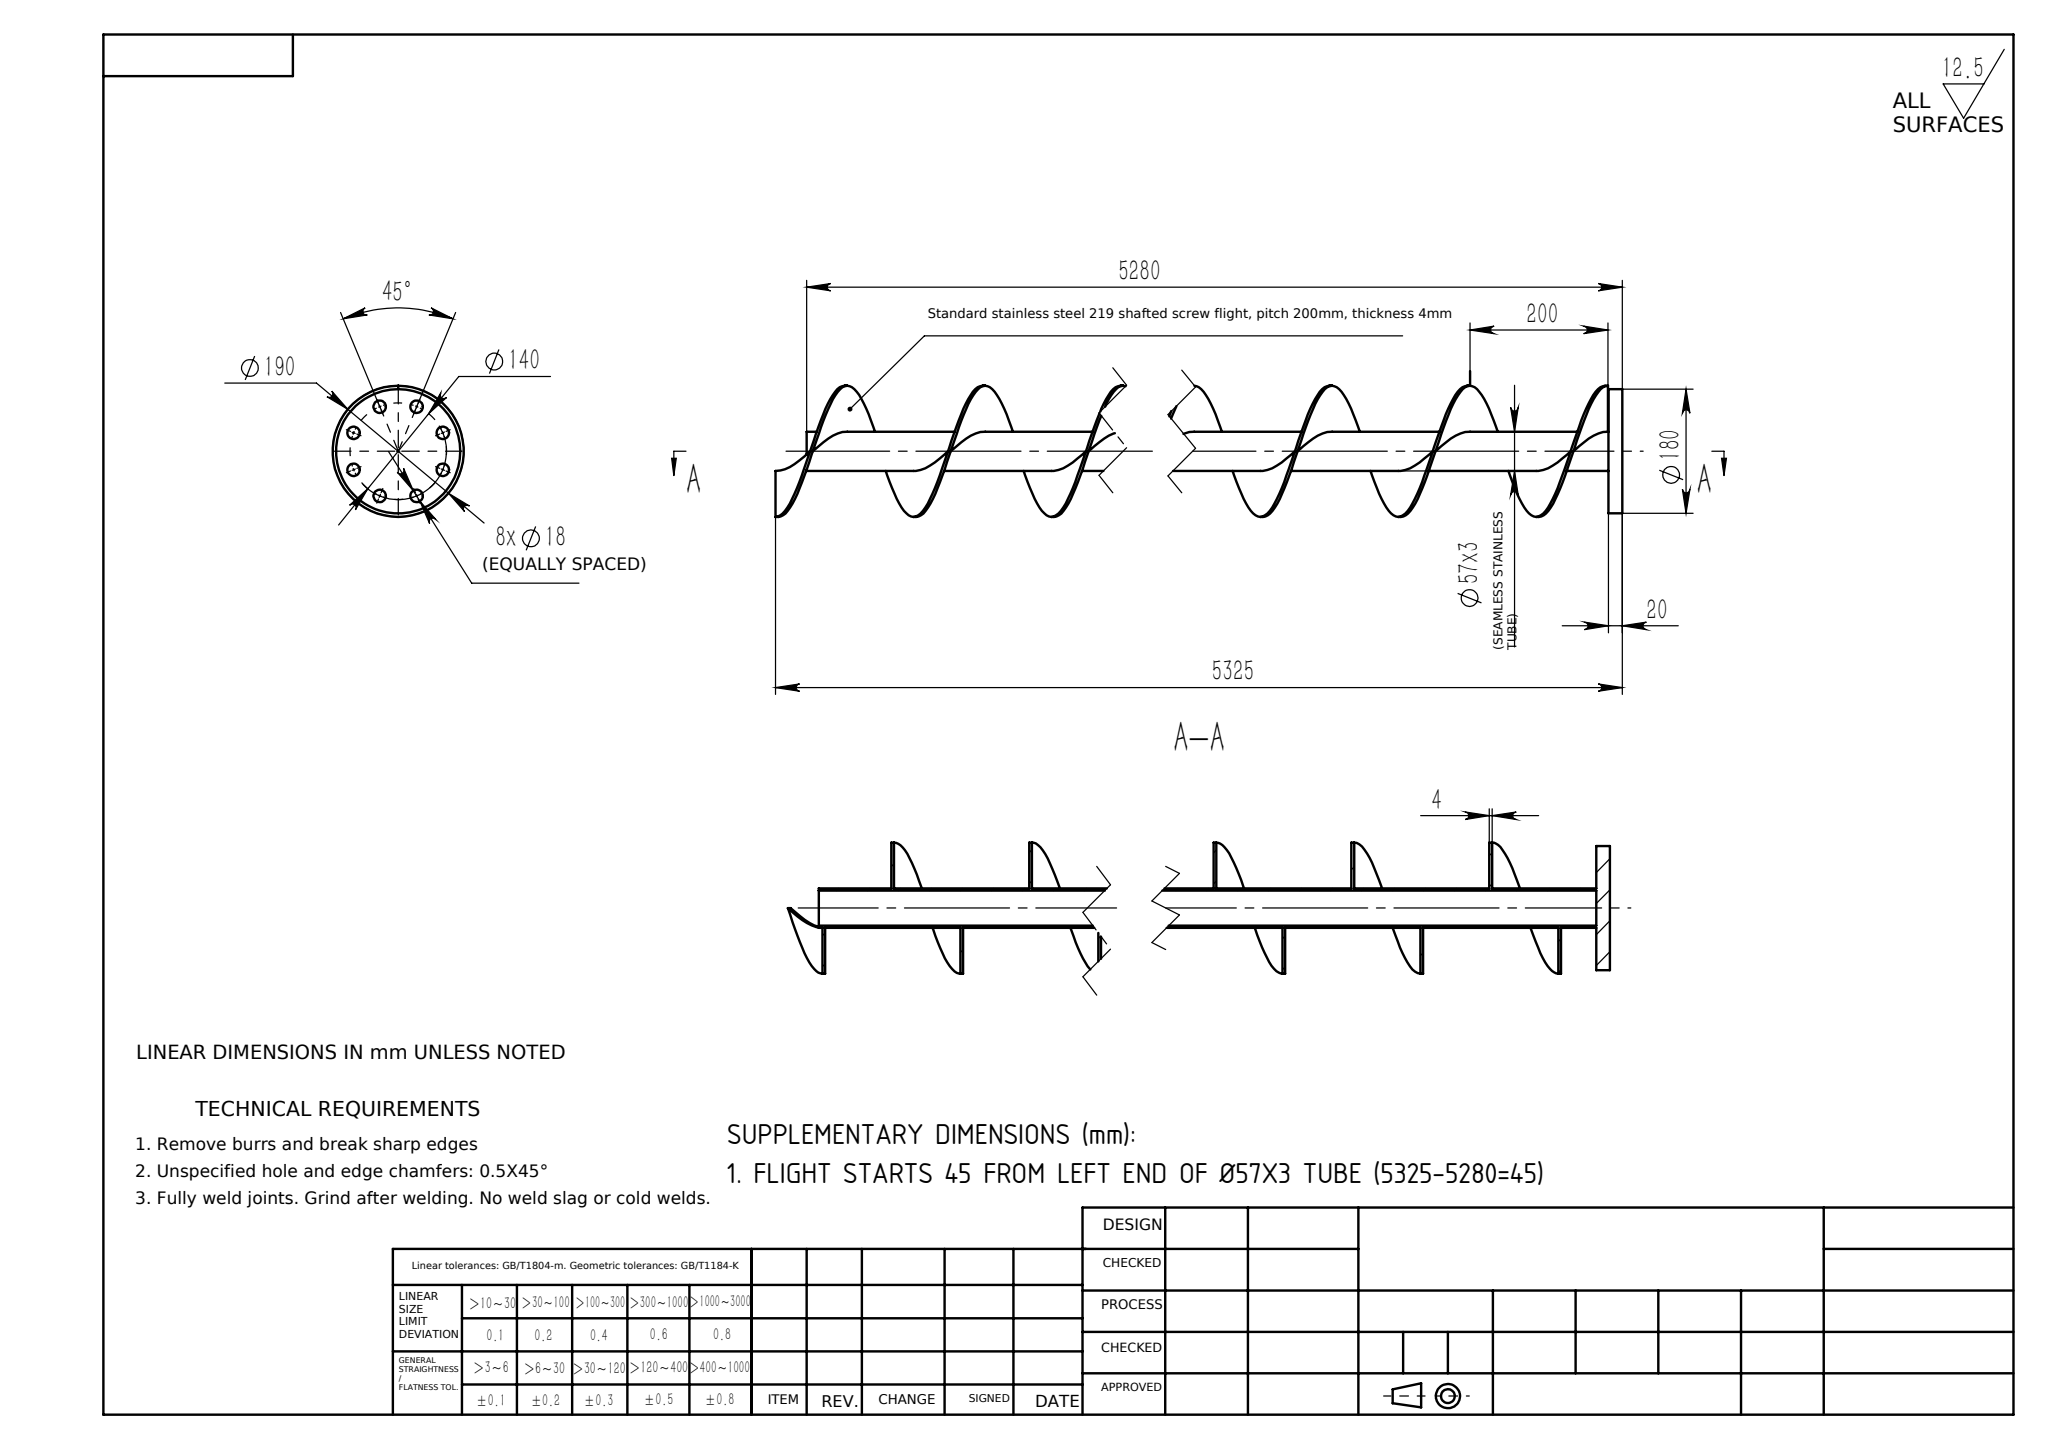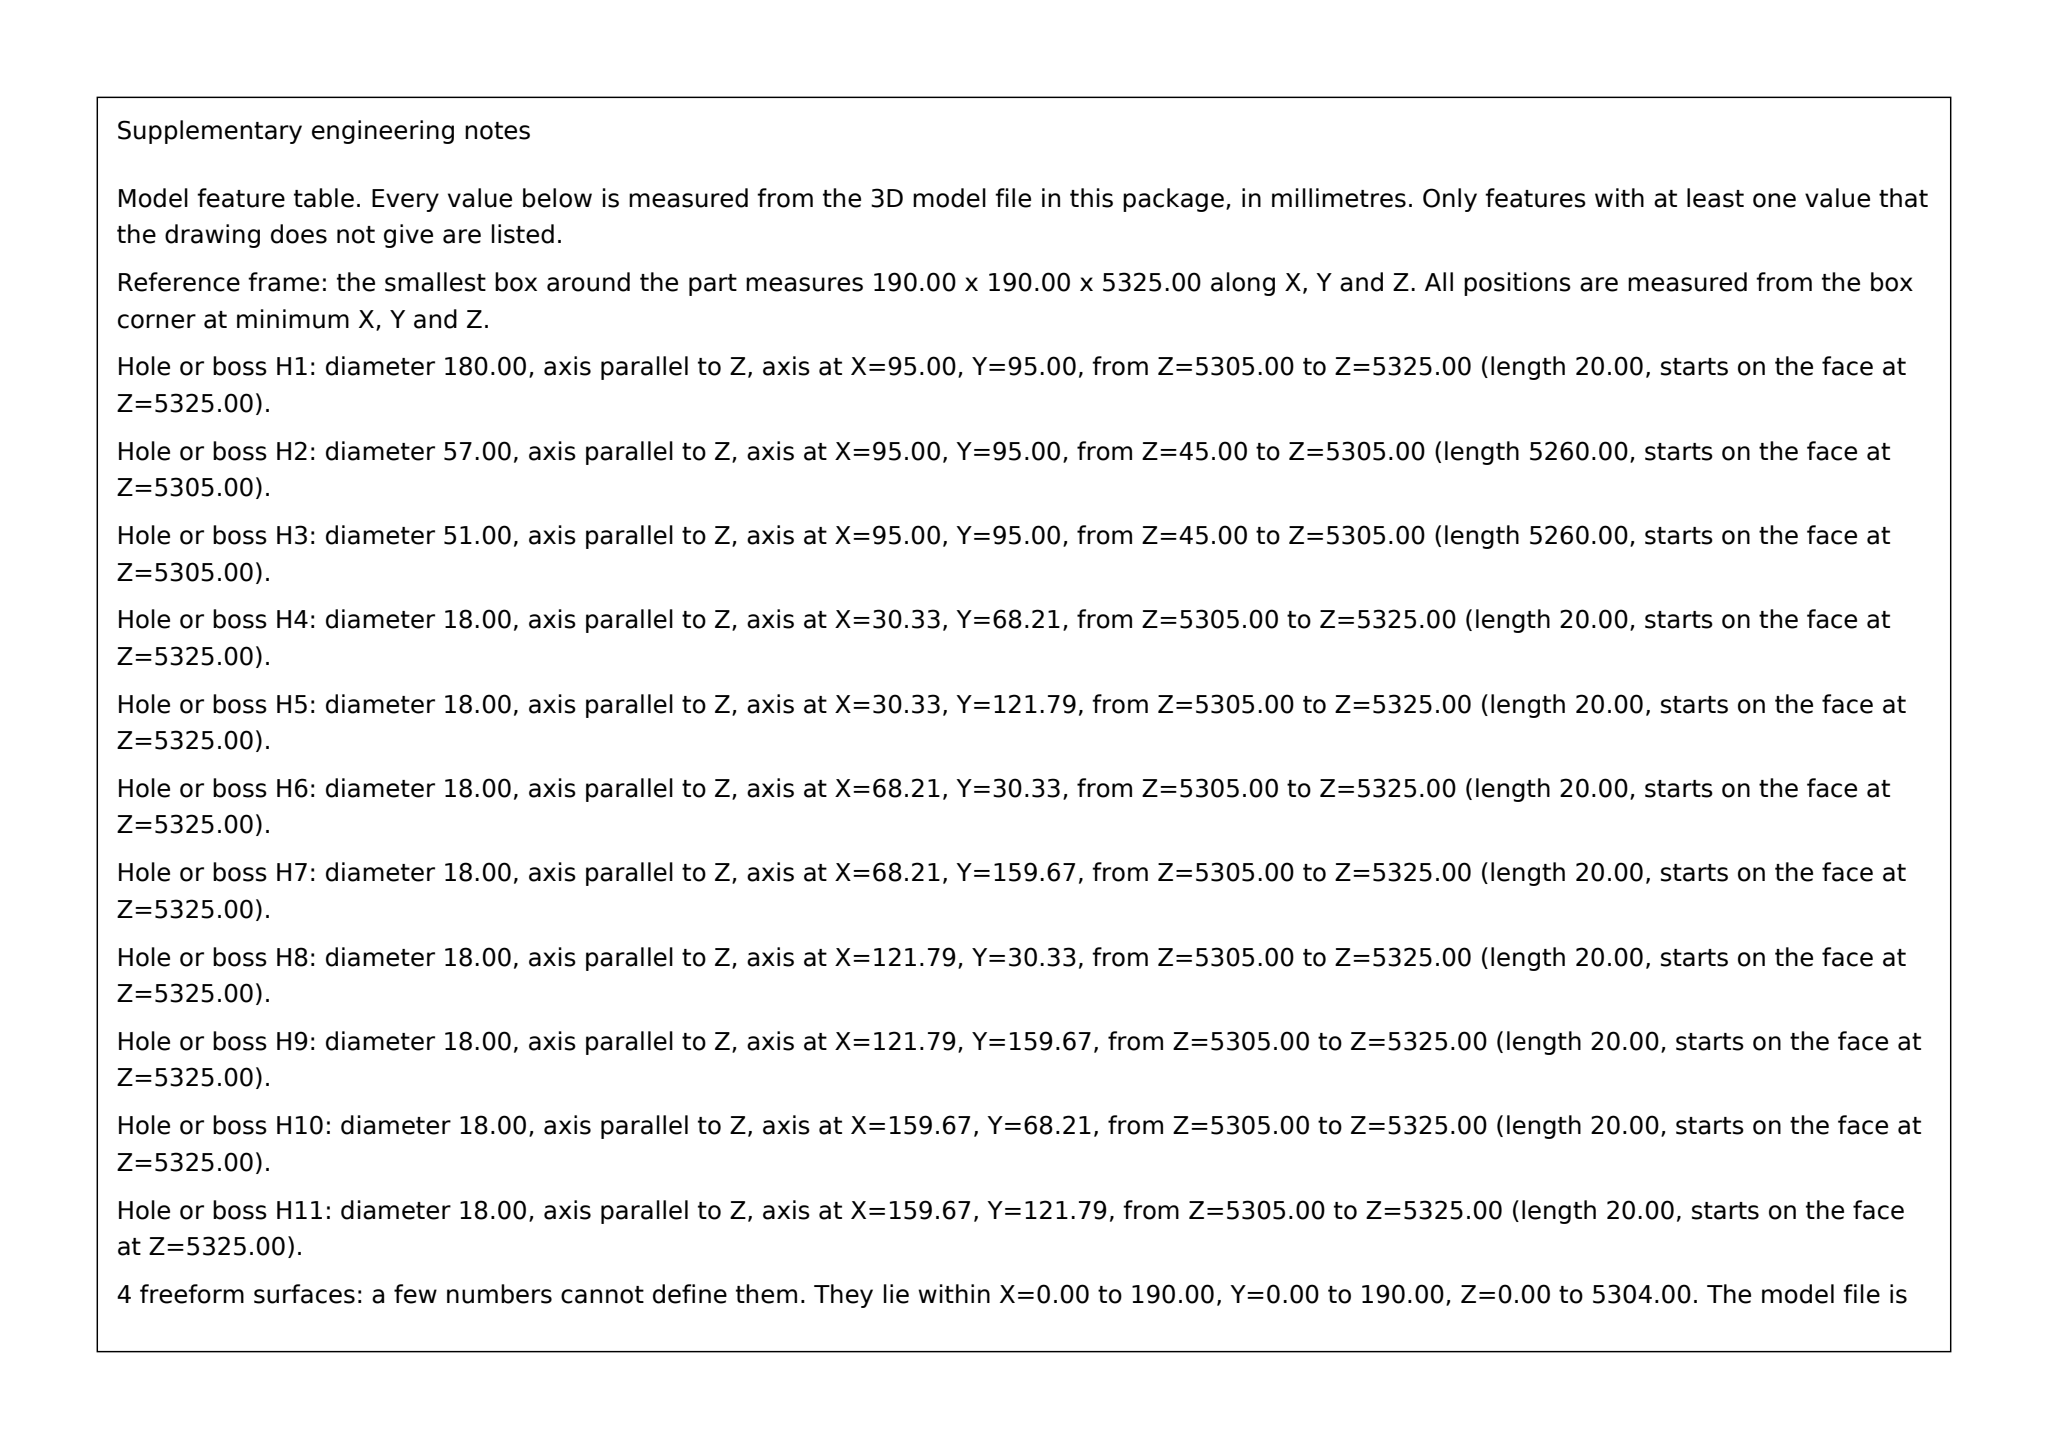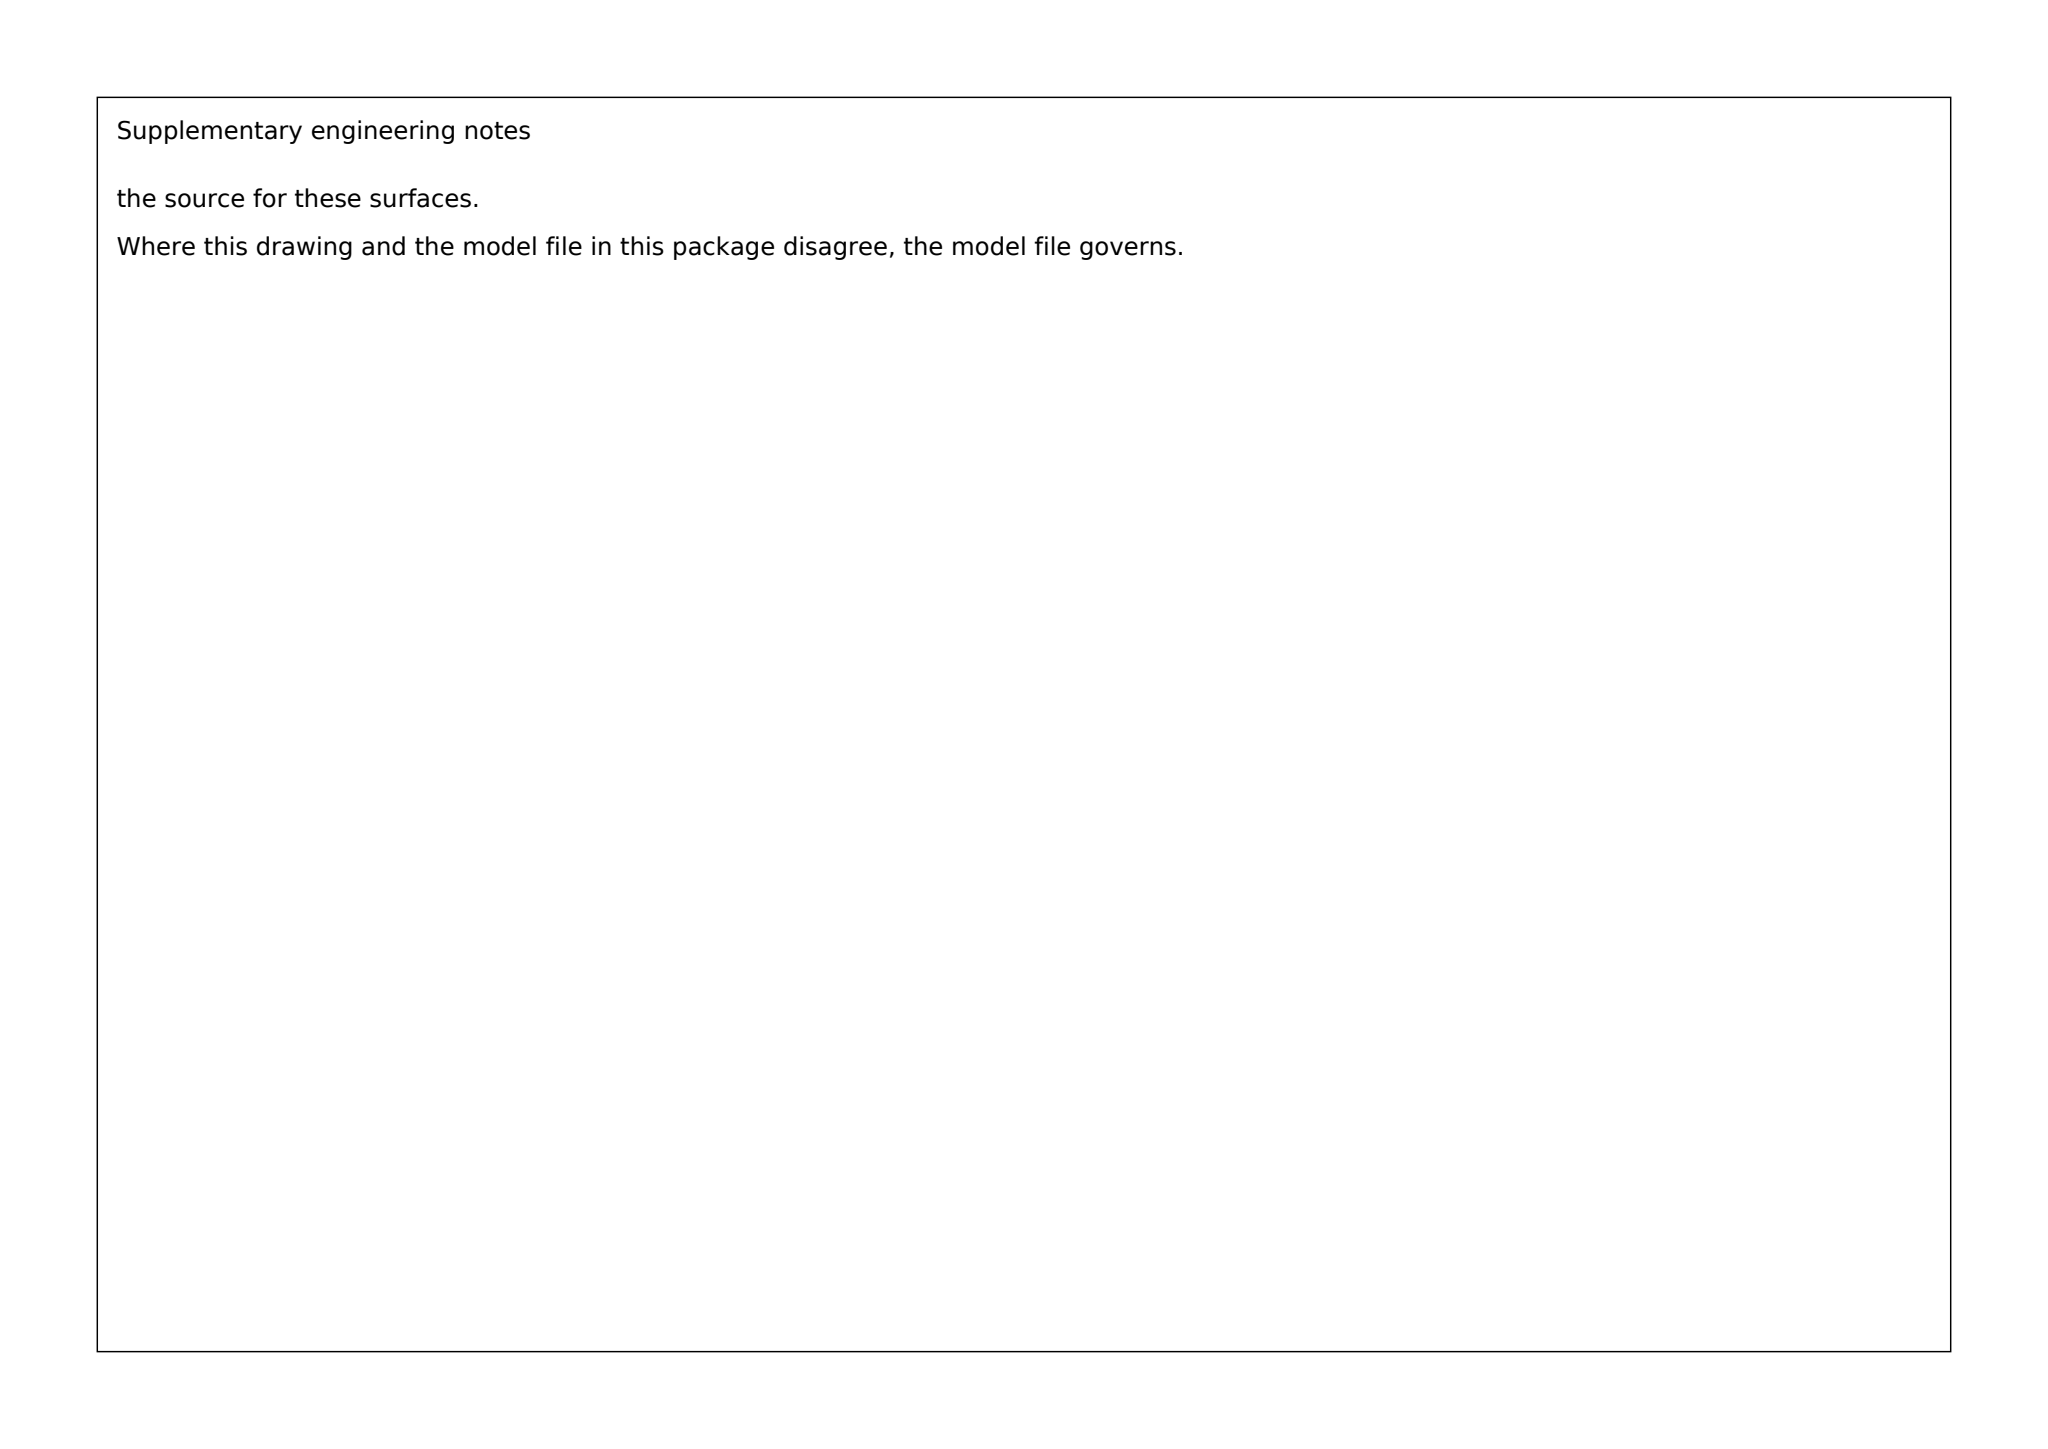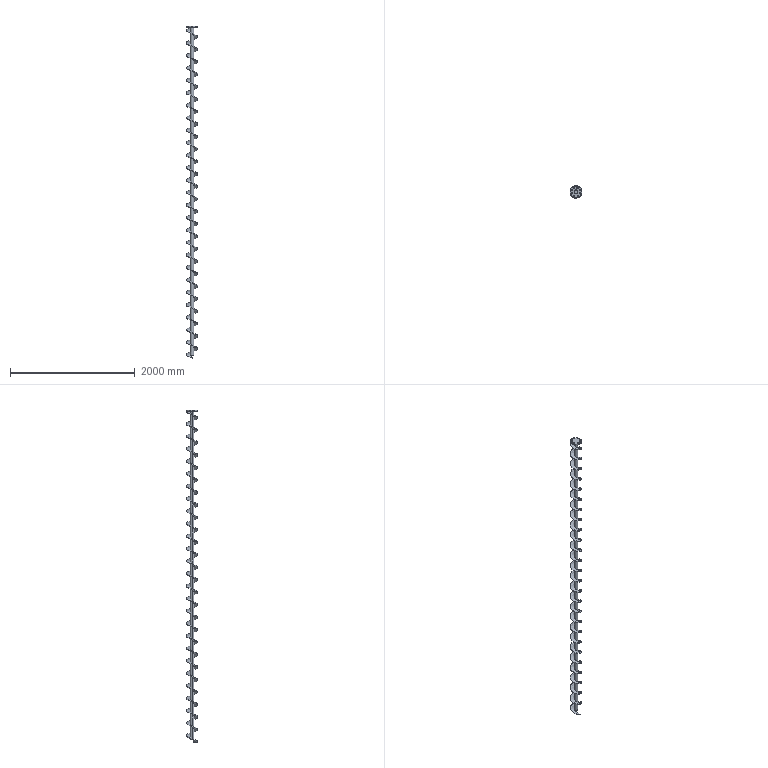Part | SolidWorks | mm | 1 solid | 85 faces | box 190 x 190 x 5325 mm | volume 5898679 mm3 | cylinder 75 | plane 6 | spline 4 | commonest cylinder face diameters 57 x55 18 x16 180 x2 51 x2